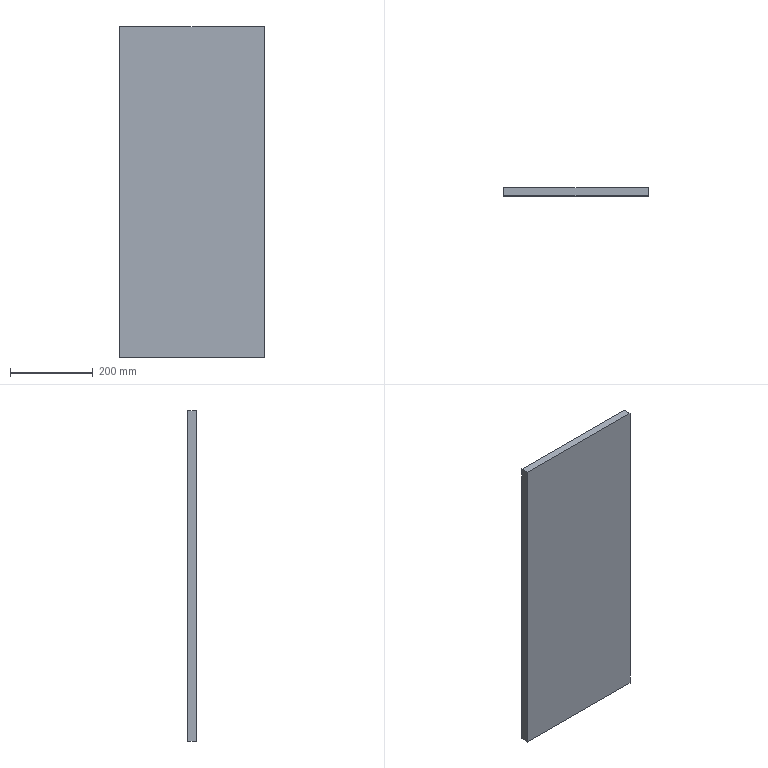Component | SolidWorks | ST60-06-1 | 1 solid | 6 faces | box 350 x 20 x 800 mm | volume 5600000 mm3 | plane 6
build123d program:
from build123d import *

# Parameters (mm, degrees)
SKETCH1_W           = 800
SKETCH1_H           = 350
BOSS_EXTRUDE1_DEPTH = 20


with BuildPart() as part:
    # Sketch1 → Boss-Extrude1 (new body)
    with BuildSketch(Plane.XY):
        with Locations((-1124.489, 541.975)):
            Rectangle(SKETCH1_W, SKETCH1_H)
    extrude(amount=BOSS_EXTRUDE1_DEPTH)


solid = part.part

# Placed as in the assembly
solid = solid.moved(Location((994.968, 135.454, -776.911), (90, 0, 90)))
STEP:
#1=CARTESIAN_POINT('',(10.945,5.333,-90.606));
#2=VERTEX_POINT('',#1);
#3=CARTESIAN_POINT('',(24.724,5.333,-90.606));
#4=VERTEX_POINT('',#3);
#5=CARTESIAN_POINT('',(10.945,5.333,-90.606));
#6=DIRECTION('',(1.,0.,0.));
#7=VECTOR('',#6,39.37);
#8=LINE('',#5,#7);
#9=EDGE_CURVE('',#2,#4,#8,.T.);
#10=ORIENTED_EDGE('',*,*,#9,.T.);
#11=CARTESIAN_POINT('',(24.724,4.545,-90.606));
#12=VERTEX_POINT('',#11);
#13=CARTESIAN_POINT('',(24.724,4.545,-90.606));
#14=DIRECTION('',(-0.,1.,-0.));
#15=VECTOR('',#14,39.37);
#16=LINE('',#13,#15);
#17=EDGE_CURVE('',#12,#4,#16,.T.);
#18=ORIENTED_EDGE('',*,*,#17,.F.);
#19=CARTESIAN_POINT('',(10.945,4.545,-90.606));
#20=VERTEX_POINT('',#19);
#21=CARTESIAN_POINT('',(10.945,4.545,-90.606));
#22=DIRECTION('',(1.,0.,0.));
#23=VECTOR('',#22,39.37);
#24=LINE('',#21,#23);
#25=EDGE_CURVE('',#20,#12,#24,.T.);
#26=ORIENTED_EDGE('',*,*,#25,.F.);
#27=CARTESIAN_POINT('',(10.945,4.545,-90.606));
#28=DIRECTION('',(-0.,1.,-0.));
#29=VECTOR('',#28,39.37);
#30=LINE('',#27,#29);
#31=EDGE_CURVE('',#20,#2,#30,.T.);
#32=ORIENTED_EDGE('',*,*,#31,.T.);
#33=EDGE_LOOP('',(#10,#18,#26,#32));
#34=FACE_OUTER_BOUND('',#33,.T.);
#35=CARTESIAN_POINT('',(10.945,4.545,-90.606));
#36=DIRECTION('',(-0.,-0.,1.));
#37=DIRECTION('',(-1.,-0.,-0.));
#38=AXIS2_PLACEMENT_3D('',#35,#36,#37);
#39=PLANE('',#38);
#40=ADVANCED_FACE('',(#34),#39,.F.);
#41=CARTESIAN_POINT('',(24.724,5.333,-59.11));
#42=VERTEX_POINT('',#41);
#43=CARTESIAN_POINT('',(24.724,5.333,-90.606));
#44=DIRECTION('',(0.,-0.,1.));
#45=VECTOR('',#44,39.37);
#46=LINE('',#43,#45);
#47=EDGE_CURVE('',#4,#42,#46,.T.);
#48=ORIENTED_EDGE('',*,*,#47,.T.);
#49=CARTESIAN_POINT('',(24.724,4.545,-59.11));
#50=VERTEX_POINT('',#49);
#51=CARTESIAN_POINT('',(24.724,4.545,-59.11));
#52=DIRECTION('',(-0.,1.,-0.));
#53=VECTOR('',#52,39.37);
#54=LINE('',#51,#53);
#55=EDGE_CURVE('',#50,#42,#54,.T.);
#56=ORIENTED_EDGE('',*,*,#55,.F.);
#57=CARTESIAN_POINT('',(24.724,4.545,-90.606));
#58=DIRECTION('',(0.,-0.,1.));
#59=VECTOR('',#58,39.37);
#60=LINE('',#57,#59);
#61=EDGE_CURVE('',#12,#50,#60,.T.);
#62=ORIENTED_EDGE('',*,*,#61,.F.);
#63=ORIENTED_EDGE('',*,*,#17,.T.);
#64=EDGE_LOOP('',(#48,#56,#62,#63));
#65=FACE_OUTER_BOUND('',#64,.T.);
#66=CARTESIAN_POINT('',(24.724,4.545,-90.606));
#67=DIRECTION('',(-1.,-0.,0.));
#68=DIRECTION('',(0.,-1.,0.));
#69=AXIS2_PLACEMENT_3D('',#66,#67,#68);
#70=PLANE('',#69);
#71=ADVANCED_FACE('',(#65),#70,.F.);
#72=CARTESIAN_POINT('',(10.945,5.333,-59.11));
#73=VERTEX_POINT('',#72);
#74=CARTESIAN_POINT('',(10.945,5.333,-59.11));
#75=DIRECTION('',(-1.,-0.,0.));
#76=VECTOR('',#75,39.37);
#77=LINE('',#74,#76);
#78=EDGE_CURVE('',#42,#73,#77,.T.);
#79=ORIENTED_EDGE('',*,*,#78,.T.);
#80=CARTESIAN_POINT('',(10.945,4.545,-59.11));
#81=VERTEX_POINT('',#80);
#82=CARTESIAN_POINT('',(10.945,4.545,-59.11));
#83=DIRECTION('',(-0.,1.,-0.));
#84=VECTOR('',#83,39.37);
#85=LINE('',#82,#84);
#86=EDGE_CURVE('',#81,#73,#85,.T.);
#87=ORIENTED_EDGE('',*,*,#86,.F.);
#88=CARTESIAN_POINT('',(10.945,4.545,-59.11));
#89=DIRECTION('',(-1.,-0.,0.));
#90=VECTOR('',#89,39.37);
#91=LINE('',#88,#90);
#92=EDGE_CURVE('',#50,#81,#91,.T.);
#93=ORIENTED_EDGE('',*,*,#92,.F.);
#94=ORIENTED_EDGE('',*,*,#55,.T.);
#95=EDGE_LOOP('',(#79,#87,#93,#94));
#96=FACE_OUTER_BOUND('',#95,.T.);
#97=CARTESIAN_POINT('',(10.945,4.545,-59.11));
#98=DIRECTION('',(-0.,-0.,-1.));
#99=DIRECTION('',(0.,-1.,0.));
#100=AXIS2_PLACEMENT_3D('',#97,#98,#99);
#101=PLANE('',#100);
#102=ADVANCED_FACE('',(#96),#101,.F.);
#103=CARTESIAN_POINT('',(10.945,5.333,-90.606));
#104=DIRECTION('',(-0.,0.,-1.));
#105=VECTOR('',#104,39.37);
#106=LINE('',#103,#105);
#107=EDGE_CURVE('',#73,#2,#106,.T.);
#108=ORIENTED_EDGE('',*,*,#107,.T.);
#109=ORIENTED_EDGE('',*,*,#31,.F.);
#110=CARTESIAN_POINT('',(10.945,4.545,-90.606));
#111=DIRECTION('',(-0.,0.,-1.));
#112=VECTOR('',#111,39.37);
#113=LINE('',#110,#112);
#114=EDGE_CURVE('',#81,#20,#113,.T.);
#115=ORIENTED_EDGE('',*,*,#114,.F.);
#116=ORIENTED_EDGE('',*,*,#86,.T.);
#117=EDGE_LOOP('',(#108,#109,#115,#116));
#118=FACE_OUTER_BOUND('',#117,.T.);
#119=CARTESIAN_POINT('',(10.945,4.545,-90.606));
#120=DIRECTION('',(1.,0.,-0.));
#121=DIRECTION('',(-0.,1.,-0.));
#122=AXIS2_PLACEMENT_3D('',#119,#120,#121);
#123=PLANE('',#122);
#124=ADVANCED_FACE('',(#118),#123,.F.);
#125=ORIENTED_EDGE('',*,*,#25,.T.);
#126=ORIENTED_EDGE('',*,*,#61,.T.);
#127=ORIENTED_EDGE('',*,*,#92,.T.);
#128=ORIENTED_EDGE('',*,*,#114,.T.);
#129=EDGE_LOOP('',(#125,#126,#127,#128));
#130=FACE_OUTER_BOUND('',#129,.T.);
#131=CARTESIAN_POINT('',(39.172,4.545,-30.587));
#132=DIRECTION('',(0.,-1.,-0.));
#133=DIRECTION('',(0.,-0.,1.));
#134=AXIS2_PLACEMENT_3D('',#131,#132,#133);
#135=PLANE('',#134);
#136=ADVANCED_FACE('',(#130),#135,.T.);
#137=ORIENTED_EDGE('',*,*,#9,.F.);
#138=ORIENTED_EDGE('',*,*,#107,.F.);
#139=ORIENTED_EDGE('',*,*,#78,.F.);
#140=ORIENTED_EDGE('',*,*,#47,.F.);
#141=EDGE_LOOP('',(#137,#138,#139,#140));
#142=FACE_OUTER_BOUND('',#141,.T.);
#143=CARTESIAN_POINT('',(39.172,5.333,-30.587));
#144=DIRECTION('',(0.,-1.,-0.));
#145=DIRECTION('',(0.,-0.,1.));
#146=AXIS2_PLACEMENT_3D('',#143,#144,#145);
#147=PLANE('',#146);
#148=ADVANCED_FACE('',(#142),#147,.F.);
#149=CLOSED_SHELL('',(#40,#71,#102,#124,#136,#148));
#150=MANIFOLD_SOLID_BREP('',#149);
#151=CARTESIAN_POINT('',(0.,0.,0.));
#152=DIRECTION('',(0.,0.,1.));
#153=DIRECTION('',(1.,0.,0.));
#154=AXIS2_PLACEMENT_3D('',#151,#152,#153);
#155=(LENGTH_UNIT()NAMED_UNIT(*)SI_UNIT($,.METRE.));
#156=LENGTH_MEASURE_WITH_UNIT(LENGTH_MEASURE(0.0254),#155);
#157=DIMENSIONAL_EXPONENTS(1.,0.,0.,0.,0.,0.,0.);
#158=(CONVERSION_BASED_UNIT('',#156)LENGTH_UNIT()NAMED_UNIT(#157));
#159=UNCERTAINTY_MEASURE_WITH_UNIT(LENGTH_MEASURE(0.00001),#158,'','');
#160=(NAMED_UNIT(*)PLANE_ANGLE_UNIT()SI_UNIT($,.RADIAN.));
#161=(NAMED_UNIT(*)SI_UNIT($,.STERADIAN.)SOLID_ANGLE_UNIT());
#162=(GEOMETRIC_REPRESENTATION_CONTEXT(3)GLOBAL_UNCERTAINTY_ASSIGNED_CONTEXT((#159))GLOBAL_UNIT_ASSIGNED_CONTEXT((#158,#160,#161))REPRESENTATION_CONTEXT('',''));
#163=ADVANCED_BREP_SHAPE_REPRESENTATION('',(#150,#154),#162);
#164=COLOUR_RGB('',0.7922,0.8196,0.9333);
#165=FILL_AREA_STYLE_COLOUR('',#164);
#166=FILL_AREA_STYLE('',(#165));
#167=SURFACE_STYLE_FILL_AREA(#166);
#168=SURFACE_SIDE_STYLE('',(#167));
#169=SURFACE_STYLE_USAGE(.BOTH.,#168);
#170=PRESENTATION_STYLE_ASSIGNMENT((#169));
#171=STYLED_ITEM('',(#170),#150);
#172=PRESENTATION_LAYER_ASSIGNMENT('','',(#171));
#173=(LENGTH_UNIT()NAMED_UNIT(*)SI_UNIT($,.METRE.));
#174=LENGTH_MEASURE_WITH_UNIT(LENGTH_MEASURE(0.0254),#173);
#175=DIMENSIONAL_EXPONENTS(1.,0.,0.,0.,0.,0.,0.);
#176=(CONVERSION_BASED_UNIT('',#174)LENGTH_UNIT()NAMED_UNIT(#175));
#177=UNCERTAINTY_MEASURE_WITH_UNIT(LENGTH_MEASURE(0.00001),#176,'','');
#178=(NAMED_UNIT(*)PLANE_ANGLE_UNIT()SI_UNIT($,.RADIAN.));
#179=(NAMED_UNIT(*)SI_UNIT($,.STERADIAN.)SOLID_ANGLE_UNIT());
#180=(GEOMETRIC_REPRESENTATION_CONTEXT(3)GLOBAL_UNCERTAINTY_ASSIGNED_CONTEXT((#177))GLOBAL_UNIT_ASSIGNED_CONTEXT((#176,#178,#179))REPRESENTATION_CONTEXT('',''));
#181=MECHANICAL_DESIGN_GEOMETRIC_PRESENTATION_REPRESENTATION('',(#171),#180);